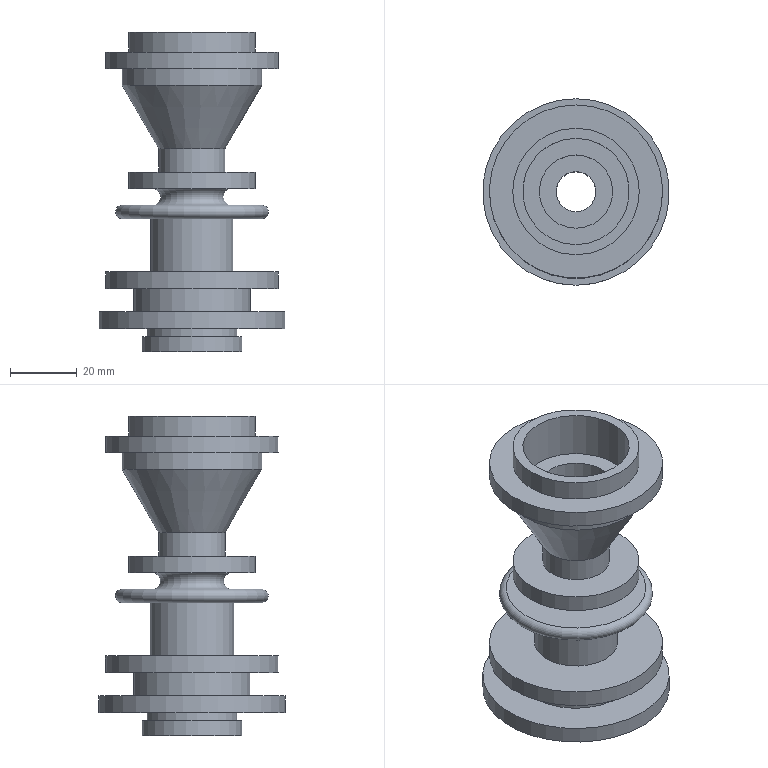Component | NX | COLUMN | 1 solid | 34 faces | volume 68351 mm3 | plane 16 | cylinder 15 | torus 2 | cone 1 | commonest cylinder face diameters 20 x2 38 x2 52 x2 12 x1 22 x1 32 x1 42 x1 25 x1